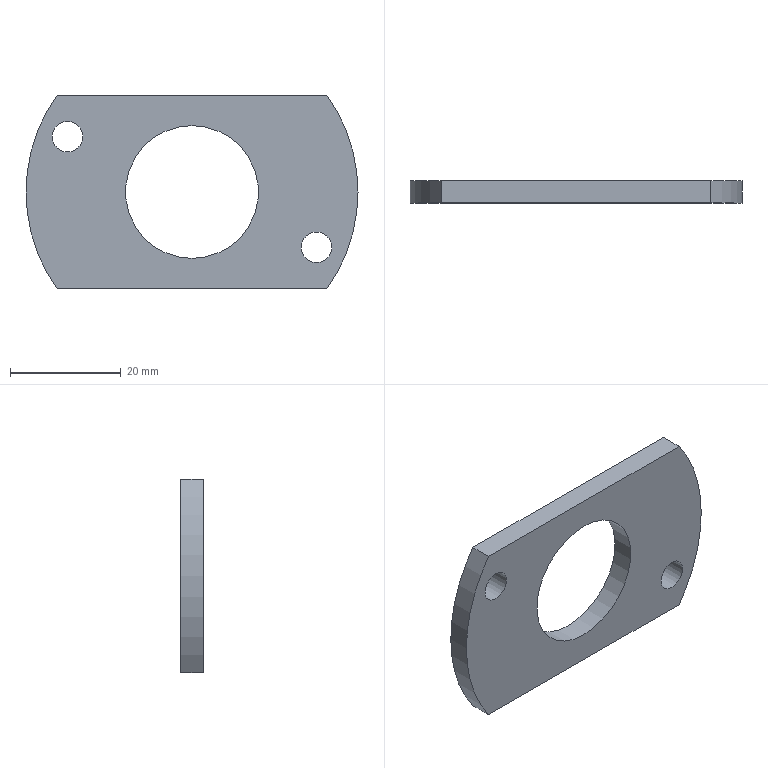Component | NX | BEARING_END_CAP_2 | 1 solid | 9 faces | box 60 x 4 x 35 mm | volume 5896 mm3 | cylinder 5 | plane 4 | commonest cylinder face diameters 60 x2 5.5 x2 24 x1
STEP:
#1=CARTESIAN_POINT('',(0.,0.,0.));
#2=DIRECTION('',(0.,0.,1.));
#3=DIRECTION('',(1.,0.,0.));
#4=AXIS2_PLACEMENT_3D('',#1,#2,#3);
#5=CARTESIAN_POINT('',(-24.367,-161.,52.5));
#6=VERTEX_POINT('',#5);
#7=CARTESIAN_POINT('',(-24.367,-161.,17.5));
#8=VERTEX_POINT('',#7);
#9=CARTESIAN_POINT('',(-0.,-161.,35.));
#10=DIRECTION('',(0.,-1.,0.));
#11=DIRECTION('',(1.,0.,0.));
#12=AXIS2_PLACEMENT_3D('',#9,#10,#11);
#13=CIRCLE('',#12,30.);
#14=CARTESIAN_POINT('',(-0.,-165.,35.));
#15=DIRECTION('',(0.,1.,0.));
#16=DIRECTION('',(0.,0.,1.));
#17=AXIS2_PLACEMENT_3D('',#14,#15,#16);
#18=CYLINDRICAL_SURFACE('',#17,30.);
#19=CARTESIAN_POINT('',(7.854,4.));
#20=DIRECTION('',(-1.,0.));
#21=VECTOR('',#20,1.);
#22=LINE('',#19,#21);
#23=(GEOMETRIC_REPRESENTATION_CONTEXT(2)PARAMETRIC_REPRESENTATION_CONTEXT()REPRESENTATION_CONTEXT('',''));
#24=DEFINITIONAL_REPRESENTATION('',(#22),#23);
#25=PCURVE('',#18,#24);
#26=CARTESIAN_POINT('',(-0.,-161.,35.));
#27=DIRECTION('',(0.,-1.,0.));
#28=DIRECTION('',(0.,0.,-1.));
#29=AXIS2_PLACEMENT_3D('',#26,#27,#28);
#30=PLANE('',#29);
#31=CARTESIAN_POINT('',(0.,0.));
#32=DIRECTION('',(0.,1.));
#33=AXIS2_PLACEMENT_2D('',#31,#32);
#34=CIRCLE('',#33,30.);
#35=(GEOMETRIC_REPRESENTATION_CONTEXT(2)PARAMETRIC_REPRESENTATION_CONTEXT()REPRESENTATION_CONTEXT('',''));
#36=DEFINITIONAL_REPRESENTATION('',(#34),#35);
#37=PCURVE('',#30,#36);
#38=SURFACE_CURVE('',#13,(#25,#37),.PCURVE_S1.);
#39=EDGE_CURVE('',#6,#8,#38,.T.);
#40=ORIENTED_EDGE('',*,*,#39,.T.);
#41=CARTESIAN_POINT('',(-24.367,-165.,17.5));
#42=VERTEX_POINT('',#41);
#43=CARTESIAN_POINT('',(-24.367,-165.,17.5));
#44=DIRECTION('',(0.,1.,0.));
#45=VECTOR('',#44,1.);
#46=LINE('',#43,#45);
#47=CARTESIAN_POINT('',(4.09,0.));
#48=DIRECTION('',(0.,1.));
#49=VECTOR('',#48,1.);
#50=LINE('',#47,#49);
#51=(GEOMETRIC_REPRESENTATION_CONTEXT(2)PARAMETRIC_REPRESENTATION_CONTEXT()REPRESENTATION_CONTEXT('',''));
#52=DEFINITIONAL_REPRESENTATION('',(#50),#51);
#53=PCURVE('',#18,#52);
#54=CARTESIAN_POINT('',(-24.367,-165.,17.5));
#55=DIRECTION('',(0.,0.,1.));
#56=DIRECTION('',(1.,0.,0.));
#57=AXIS2_PLACEMENT_3D('',#54,#55,#56);
#58=PLANE('',#57);
#59=CARTESIAN_POINT('',(0.,0.));
#60=DIRECTION('',(0.,1.));
#61=VECTOR('',#60,1.);
#62=LINE('',#59,#61);
#63=(GEOMETRIC_REPRESENTATION_CONTEXT(2)PARAMETRIC_REPRESENTATION_CONTEXT()REPRESENTATION_CONTEXT('',''));
#64=DEFINITIONAL_REPRESENTATION('',(#62),#63);
#65=PCURVE('',#58,#64);
#66=SURFACE_CURVE('',#46,(#53,#65),.PCURVE_S1.);
#67=EDGE_CURVE('',#42,#8,#66,.T.);
#68=ORIENTED_EDGE('',*,*,#67,.F.);
#69=CARTESIAN_POINT('',(-24.367,-165.,52.5));
#70=VERTEX_POINT('',#69);
#71=CARTESIAN_POINT('',(-0.,-165.,35.));
#72=DIRECTION('',(0.,-1.,0.));
#73=DIRECTION('',(1.,0.,0.));
#74=AXIS2_PLACEMENT_3D('',#71,#72,#73);
#75=CIRCLE('',#74,30.);
#76=CARTESIAN_POINT('',(7.854,0.));
#77=DIRECTION('',(-1.,0.));
#78=VECTOR('',#77,1.);
#79=LINE('',#76,#78);
#80=(GEOMETRIC_REPRESENTATION_CONTEXT(2)PARAMETRIC_REPRESENTATION_CONTEXT()REPRESENTATION_CONTEXT('',''));
#81=DEFINITIONAL_REPRESENTATION('',(#79),#80);
#82=PCURVE('',#18,#81);
#83=CARTESIAN_POINT('',(-0.,-165.,35.));
#84=DIRECTION('',(0.,-1.,0.));
#85=DIRECTION('',(0.,0.,-1.));
#86=AXIS2_PLACEMENT_3D('',#83,#84,#85);
#87=PLANE('',#86);
#88=CARTESIAN_POINT('',(0.,0.));
#89=DIRECTION('',(0.,1.));
#90=AXIS2_PLACEMENT_2D('',#88,#89);
#91=CIRCLE('',#90,30.);
#92=(GEOMETRIC_REPRESENTATION_CONTEXT(2)PARAMETRIC_REPRESENTATION_CONTEXT()REPRESENTATION_CONTEXT('',''));
#93=DEFINITIONAL_REPRESENTATION('',(#91),#92);
#94=PCURVE('',#87,#93);
#95=SURFACE_CURVE('',#75,(#82,#94),.PCURVE_S1.);
#96=EDGE_CURVE('',#70,#42,#95,.T.);
#97=ORIENTED_EDGE('',*,*,#96,.F.);
#98=CARTESIAN_POINT('',(-24.367,-165.,52.5));
#99=DIRECTION('',(0.,1.,0.));
#100=VECTOR('',#99,1.);
#101=LINE('',#98,#100);
#102=CARTESIAN_POINT('',(5.335,0.));
#103=DIRECTION('',(0.,1.));
#104=VECTOR('',#103,1.);
#105=LINE('',#102,#104);
#106=(GEOMETRIC_REPRESENTATION_CONTEXT(2)PARAMETRIC_REPRESENTATION_CONTEXT()REPRESENTATION_CONTEXT('',''));
#107=DEFINITIONAL_REPRESENTATION('',(#105),#106);
#108=PCURVE('',#18,#107);
#109=CARTESIAN_POINT('',(24.367,-165.,52.5));
#110=DIRECTION('',(0.,0.,-1.));
#111=DIRECTION('',(-1.,0.,0.));
#112=AXIS2_PLACEMENT_3D('',#109,#110,#111);
#113=PLANE('',#112);
#114=CARTESIAN_POINT('',(48.734,0.));
#115=DIRECTION('',(0.,1.));
#116=VECTOR('',#115,1.);
#117=LINE('',#114,#116);
#118=(GEOMETRIC_REPRESENTATION_CONTEXT(2)PARAMETRIC_REPRESENTATION_CONTEXT()REPRESENTATION_CONTEXT('',''));
#119=DEFINITIONAL_REPRESENTATION('',(#117),#118);
#120=PCURVE('',#113,#119);
#121=SURFACE_CURVE('',#101,(#108,#120),.PCURVE_S1.);
#122=EDGE_CURVE('',#70,#6,#121,.T.);
#123=ORIENTED_EDGE('',*,*,#122,.T.);
#124=EDGE_LOOP('',(#40,#68,#97,#123));
#125=FACE_BOUND('',#124,.T.);
#126=ADVANCED_FACE('',(#125),#18,.T.);
#127=CARTESIAN_POINT('',(24.367,-161.,17.5));
#128=VERTEX_POINT('',#127);
#129=CARTESIAN_POINT('',(-24.367,-161.,17.5));
#130=DIRECTION('',(1.,0.,0.));
#131=VECTOR('',#130,1.);
#132=LINE('',#129,#131);
#133=CARTESIAN_POINT('',(0.,4.));
#134=DIRECTION('',(1.,0.));
#135=VECTOR('',#134,1.);
#136=LINE('',#133,#135);
#137=(GEOMETRIC_REPRESENTATION_CONTEXT(2)PARAMETRIC_REPRESENTATION_CONTEXT()REPRESENTATION_CONTEXT('',''));
#138=DEFINITIONAL_REPRESENTATION('',(#136),#137);
#139=PCURVE('',#58,#138);
#140=CARTESIAN_POINT('',(17.5,-24.367));
#141=DIRECTION('',(0.,1.));
#142=VECTOR('',#141,1.);
#143=LINE('',#140,#142);
#144=(GEOMETRIC_REPRESENTATION_CONTEXT(2)PARAMETRIC_REPRESENTATION_CONTEXT()REPRESENTATION_CONTEXT('',''));
#145=DEFINITIONAL_REPRESENTATION('',(#143),#144);
#146=PCURVE('',#30,#145);
#147=SURFACE_CURVE('',#132,(#139,#146),.PCURVE_S1.);
#148=EDGE_CURVE('',#8,#128,#147,.T.);
#149=ORIENTED_EDGE('',*,*,#148,.T.);
#150=CARTESIAN_POINT('',(24.367,-165.,17.5));
#151=VERTEX_POINT('',#150);
#152=CARTESIAN_POINT('',(24.367,-165.,17.5));
#153=DIRECTION('',(0.,1.,0.));
#154=VECTOR('',#153,1.);
#155=LINE('',#152,#154);
#156=CARTESIAN_POINT('',(48.734,0.));
#157=DIRECTION('',(0.,1.));
#158=VECTOR('',#157,1.);
#159=LINE('',#156,#158);
#160=(GEOMETRIC_REPRESENTATION_CONTEXT(2)PARAMETRIC_REPRESENTATION_CONTEXT()REPRESENTATION_CONTEXT('',''));
#161=DEFINITIONAL_REPRESENTATION('',(#159),#160);
#162=PCURVE('',#58,#161);
#163=CARTESIAN_POINT('',(-0.,-165.,35.));
#164=DIRECTION('',(0.,1.,0.));
#165=DIRECTION('',(0.,0.,1.));
#166=AXIS2_PLACEMENT_3D('',#163,#164,#165);
#167=CYLINDRICAL_SURFACE('',#166,30.);
#168=CARTESIAN_POINT('',(2.194,0.));
#169=DIRECTION('',(0.,1.));
#170=VECTOR('',#169,1.);
#171=LINE('',#168,#170);
#172=(GEOMETRIC_REPRESENTATION_CONTEXT(2)PARAMETRIC_REPRESENTATION_CONTEXT()REPRESENTATION_CONTEXT('',''));
#173=DEFINITIONAL_REPRESENTATION('',(#171),#172);
#174=PCURVE('',#167,#173);
#175=SURFACE_CURVE('',#155,(#162,#174),.PCURVE_S1.);
#176=EDGE_CURVE('',#151,#128,#175,.T.);
#177=ORIENTED_EDGE('',*,*,#176,.F.);
#178=CARTESIAN_POINT('',(-24.367,-165.,17.5));
#179=DIRECTION('',(1.,0.,0.));
#180=VECTOR('',#179,1.);
#181=LINE('',#178,#180);
#182=CARTESIAN_POINT('',(0.,0.));
#183=DIRECTION('',(1.,0.));
#184=VECTOR('',#183,1.);
#185=LINE('',#182,#184);
#186=(GEOMETRIC_REPRESENTATION_CONTEXT(2)PARAMETRIC_REPRESENTATION_CONTEXT()REPRESENTATION_CONTEXT('',''));
#187=DEFINITIONAL_REPRESENTATION('',(#185),#186);
#188=PCURVE('',#58,#187);
#189=CARTESIAN_POINT('',(17.5,-24.367));
#190=DIRECTION('',(0.,1.));
#191=VECTOR('',#190,1.);
#192=LINE('',#189,#191);
#193=(GEOMETRIC_REPRESENTATION_CONTEXT(2)PARAMETRIC_REPRESENTATION_CONTEXT()REPRESENTATION_CONTEXT('',''));
#194=DEFINITIONAL_REPRESENTATION('',(#192),#193);
#195=PCURVE('',#87,#194);
#196=SURFACE_CURVE('',#181,(#188,#195),.PCURVE_S1.);
#197=EDGE_CURVE('',#42,#151,#196,.T.);
#198=ORIENTED_EDGE('',*,*,#197,.F.);
#199=ORIENTED_EDGE('',*,*,#67,.T.);
#200=EDGE_LOOP('',(#149,#177,#198,#199));
#201=FACE_BOUND('',#200,.T.);
#202=ADVANCED_FACE('',(#201),#58,.F.);
#203=CARTESIAN_POINT('',(24.367,-161.,52.5));
#204=VERTEX_POINT('',#203);
#205=CARTESIAN_POINT('',(-0.,-161.,35.));
#206=DIRECTION('',(0.,-1.,0.));
#207=DIRECTION('',(1.,0.,0.));
#208=AXIS2_PLACEMENT_3D('',#205,#206,#207);
#209=CIRCLE('',#208,30.);
#210=CARTESIAN_POINT('',(7.854,4.));
#211=DIRECTION('',(-1.,0.));
#212=VECTOR('',#211,1.);
#213=LINE('',#210,#212);
#214=(GEOMETRIC_REPRESENTATION_CONTEXT(2)PARAMETRIC_REPRESENTATION_CONTEXT()REPRESENTATION_CONTEXT('',''));
#215=DEFINITIONAL_REPRESENTATION('',(#213),#214);
#216=PCURVE('',#167,#215);
#217=CARTESIAN_POINT('',(0.,0.));
#218=DIRECTION('',(0.,1.));
#219=AXIS2_PLACEMENT_2D('',#217,#218);
#220=CIRCLE('',#219,30.);
#221=(GEOMETRIC_REPRESENTATION_CONTEXT(2)PARAMETRIC_REPRESENTATION_CONTEXT()REPRESENTATION_CONTEXT('',''));
#222=DEFINITIONAL_REPRESENTATION('',(#220),#221);
#223=PCURVE('',#30,#222);
#224=SURFACE_CURVE('',#209,(#216,#223),.PCURVE_S1.);
#225=EDGE_CURVE('',#128,#204,#224,.T.);
#226=ORIENTED_EDGE('',*,*,#225,.T.);
#227=CARTESIAN_POINT('',(24.367,-165.,52.5));
#228=VERTEX_POINT('',#227);
#229=CARTESIAN_POINT('',(24.367,-165.,52.5));
#230=DIRECTION('',(0.,1.,0.));
#231=VECTOR('',#230,1.);
#232=LINE('',#229,#231);
#233=CARTESIAN_POINT('',(0.948,0.));
#234=DIRECTION('',(0.,1.));
#235=VECTOR('',#234,1.);
#236=LINE('',#233,#235);
#237=(GEOMETRIC_REPRESENTATION_CONTEXT(2)PARAMETRIC_REPRESENTATION_CONTEXT()REPRESENTATION_CONTEXT('',''));
#238=DEFINITIONAL_REPRESENTATION('',(#236),#237);
#239=PCURVE('',#167,#238);
#240=CARTESIAN_POINT('',(-0.,0.));
#241=DIRECTION('',(0.,1.));
#242=VECTOR('',#241,1.);
#243=LINE('',#240,#242);
#244=(GEOMETRIC_REPRESENTATION_CONTEXT(2)PARAMETRIC_REPRESENTATION_CONTEXT()REPRESENTATION_CONTEXT('',''));
#245=DEFINITIONAL_REPRESENTATION('',(#243),#244);
#246=PCURVE('',#113,#245);
#247=SURFACE_CURVE('',#232,(#239,#246),.PCURVE_S1.);
#248=EDGE_CURVE('',#228,#204,#247,.T.);
#249=ORIENTED_EDGE('',*,*,#248,.F.);
#250=CARTESIAN_POINT('',(-0.,-165.,35.));
#251=DIRECTION('',(0.,-1.,0.));
#252=DIRECTION('',(1.,0.,0.));
#253=AXIS2_PLACEMENT_3D('',#250,#251,#252);
#254=CIRCLE('',#253,30.);
#255=CARTESIAN_POINT('',(7.854,0.));
#256=DIRECTION('',(-1.,0.));
#257=VECTOR('',#256,1.);
#258=LINE('',#255,#257);
#259=(GEOMETRIC_REPRESENTATION_CONTEXT(2)PARAMETRIC_REPRESENTATION_CONTEXT()REPRESENTATION_CONTEXT('',''));
#260=DEFINITIONAL_REPRESENTATION('',(#258),#259);
#261=PCURVE('',#167,#260);
#262=CARTESIAN_POINT('',(0.,0.));
#263=DIRECTION('',(0.,1.));
#264=AXIS2_PLACEMENT_2D('',#262,#263);
#265=CIRCLE('',#264,30.);
#266=(GEOMETRIC_REPRESENTATION_CONTEXT(2)PARAMETRIC_REPRESENTATION_CONTEXT()REPRESENTATION_CONTEXT('',''));
#267=DEFINITIONAL_REPRESENTATION('',(#265),#266);
#268=PCURVE('',#87,#267);
#269=SURFACE_CURVE('',#254,(#261,#268),.PCURVE_S1.);
#270=EDGE_CURVE('',#151,#228,#269,.T.);
#271=ORIENTED_EDGE('',*,*,#270,.F.);
#272=ORIENTED_EDGE('',*,*,#176,.T.);
#273=EDGE_LOOP('',(#226,#249,#271,#272));
#274=FACE_BOUND('',#273,.T.);
#275=ADVANCED_FACE('',(#274),#167,.T.);
#276=CARTESIAN_POINT('',(24.367,-161.,52.5));
#277=DIRECTION('',(-1.,0.,0.));
#278=VECTOR('',#277,1.);
#279=LINE('',#276,#278);
#280=CARTESIAN_POINT('',(0.,4.));
#281=DIRECTION('',(1.,0.));
#282=VECTOR('',#281,1.);
#283=LINE('',#280,#282);
#284=(GEOMETRIC_REPRESENTATION_CONTEXT(2)PARAMETRIC_REPRESENTATION_CONTEXT()REPRESENTATION_CONTEXT('',''));
#285=DEFINITIONAL_REPRESENTATION('',(#283),#284);
#286=PCURVE('',#113,#285);
#287=CARTESIAN_POINT('',(-17.5,24.367));
#288=DIRECTION('',(0.,-1.));
#289=VECTOR('',#288,1.);
#290=LINE('',#287,#289);
#291=(GEOMETRIC_REPRESENTATION_CONTEXT(2)PARAMETRIC_REPRESENTATION_CONTEXT()REPRESENTATION_CONTEXT('',''));
#292=DEFINITIONAL_REPRESENTATION('',(#290),#291);
#293=PCURVE('',#30,#292);
#294=SURFACE_CURVE('',#279,(#286,#293),.PCURVE_S1.);
#295=EDGE_CURVE('',#204,#6,#294,.T.);
#296=ORIENTED_EDGE('',*,*,#295,.T.);
#297=ORIENTED_EDGE('',*,*,#122,.F.);
#298=CARTESIAN_POINT('',(24.367,-165.,52.5));
#299=DIRECTION('',(-1.,0.,0.));
#300=VECTOR('',#299,1.);
#301=LINE('',#298,#300);
#302=CARTESIAN_POINT('',(0.,0.));
#303=DIRECTION('',(1.,0.));
#304=VECTOR('',#303,1.);
#305=LINE('',#302,#304);
#306=(GEOMETRIC_REPRESENTATION_CONTEXT(2)PARAMETRIC_REPRESENTATION_CONTEXT()REPRESENTATION_CONTEXT('',''));
#307=DEFINITIONAL_REPRESENTATION('',(#305),#306);
#308=PCURVE('',#113,#307);
#309=CARTESIAN_POINT('',(-17.5,24.367));
#310=DIRECTION('',(0.,-1.));
#311=VECTOR('',#310,1.);
#312=LINE('',#309,#311);
#313=(GEOMETRIC_REPRESENTATION_CONTEXT(2)PARAMETRIC_REPRESENTATION_CONTEXT()REPRESENTATION_CONTEXT('',''));
#314=DEFINITIONAL_REPRESENTATION('',(#312),#313);
#315=PCURVE('',#87,#314);
#316=SURFACE_CURVE('',#301,(#308,#315),.PCURVE_S1.);
#317=EDGE_CURVE('',#228,#70,#316,.T.);
#318=ORIENTED_EDGE('',*,*,#317,.F.);
#319=ORIENTED_EDGE('',*,*,#248,.T.);
#320=EDGE_LOOP('',(#296,#297,#318,#319));
#321=FACE_BOUND('',#320,.T.);
#322=ADVANCED_FACE('',(#321),#113,.F.);
#323=CARTESIAN_POINT('',(22.5,-165.,27.75));
#324=VERTEX_POINT('',#323);
#325=CARTESIAN_POINT('',(22.5,-165.,25.));
#326=DIRECTION('',(0.,1.,0.));
#327=DIRECTION('',(0.,0.,1.));
#328=AXIS2_PLACEMENT_3D('',#325,#326,#327);
#329=CIRCLE('',#328,2.75);
#330=CARTESIAN_POINT('',(7.25,22.5));
#331=CARTESIAN_POINT('',(7.25,27.263));
#332=CARTESIAN_POINT('',(11.375,24.882));
#333=CARTESIAN_POINT('',(15.5,22.5));
#334=CARTESIAN_POINT('',(11.375,20.118));
#335=CARTESIAN_POINT('',(7.25,17.737));
#336=CARTESIAN_POINT('',(7.25,22.5));
#337=(BOUNDED_CURVE()B_SPLINE_CURVE(2,(#330,#331,#332,#333,#334,#335,#336),.UNSPECIFIED.,.T.,.F.)B_SPLINE_CURVE_WITH_KNOTS((1,2,2,2,2,1),(-2.094,0.,2.094,4.189,6.283,8.378),.UNSPECIFIED.)CURVE()GEOMETRIC_REPRESENTATION_ITEM()RATIONAL_B_SPLINE_CURVE((1.,0.5,1.,0.5,1.,0.5,1.))REPRESENTATION_ITEM(''));
#338=(GEOMETRIC_REPRESENTATION_CONTEXT(2)PARAMETRIC_REPRESENTATION_CONTEXT()REPRESENTATION_CONTEXT('',''));
#339=DEFINITIONAL_REPRESENTATION('',(#337),#338);
#340=PCURVE('',#87,#339);
#341=CARTESIAN_POINT('',(22.5,-165.,25.));
#342=DIRECTION('',(0.,1.,0.));
#343=DIRECTION('',(0.,0.,1.));
#344=AXIS2_PLACEMENT_3D('',#341,#342,#343);
#345=CYLINDRICAL_SURFACE('',#344,2.75);
#346=CARTESIAN_POINT('',(0.,0.));
#347=DIRECTION('',(1.,0.));
#348=VECTOR('',#347,1.);
#349=LINE('',#346,#348);
#350=(GEOMETRIC_REPRESENTATION_CONTEXT(2)PARAMETRIC_REPRESENTATION_CONTEXT()REPRESENTATION_CONTEXT('',''));
#351=DEFINITIONAL_REPRESENTATION('',(#349),#350);
#352=PCURVE('',#345,#351);
#353=SURFACE_CURVE('',#329,(#340,#352),.PCURVE_S1.);
#354=EDGE_CURVE('',#324,#324,#353,.T.);
#355=ORIENTED_EDGE('',*,*,#354,.T.);
#356=EDGE_LOOP('',(#355));
#357=FACE_BOUND('',#356,.T.);
#358=CARTESIAN_POINT('',(-22.5,-165.,47.75));
#359=VERTEX_POINT('',#358);
#360=CARTESIAN_POINT('',(-22.5,-165.,45.));
#361=DIRECTION('',(0.,1.,0.));
#362=DIRECTION('',(0.,0.,1.));
#363=AXIS2_PLACEMENT_3D('',#360,#361,#362);
#364=CIRCLE('',#363,2.75);
#365=CARTESIAN_POINT('',(-12.75,-22.5));
#366=CARTESIAN_POINT('',(-12.75,-17.737));
#367=CARTESIAN_POINT('',(-8.625,-20.118));
#368=CARTESIAN_POINT('',(-4.5,-22.5));
#369=CARTESIAN_POINT('',(-8.625,-24.882));
#370=CARTESIAN_POINT('',(-12.75,-27.263));
#371=CARTESIAN_POINT('',(-12.75,-22.5));
#372=(BOUNDED_CURVE()B_SPLINE_CURVE(2,(#365,#366,#367,#368,#369,#370,#371),.UNSPECIFIED.,.T.,.F.)B_SPLINE_CURVE_WITH_KNOTS((1,2,2,2,2,1),(-2.094,0.,2.094,4.189,6.283,8.378),.UNSPECIFIED.)CURVE()GEOMETRIC_REPRESENTATION_ITEM()RATIONAL_B_SPLINE_CURVE((1.,0.5,1.,0.5,1.,0.5,1.))REPRESENTATION_ITEM(''));
#373=(GEOMETRIC_REPRESENTATION_CONTEXT(2)PARAMETRIC_REPRESENTATION_CONTEXT()REPRESENTATION_CONTEXT('',''));
#374=DEFINITIONAL_REPRESENTATION('',(#372),#373);
#375=PCURVE('',#87,#374);
#376=CARTESIAN_POINT('',(-22.5,-165.,45.));
#377=DIRECTION('',(0.,1.,0.));
#378=DIRECTION('',(0.,0.,1.));
#379=AXIS2_PLACEMENT_3D('',#376,#377,#378);
#380=CYLINDRICAL_SURFACE('',#379,2.75);
#381=CARTESIAN_POINT('',(0.,0.));
#382=DIRECTION('',(1.,0.));
#383=VECTOR('',#382,1.);
#384=LINE('',#381,#383);
#385=(GEOMETRIC_REPRESENTATION_CONTEXT(2)PARAMETRIC_REPRESENTATION_CONTEXT()REPRESENTATION_CONTEXT('',''));
#386=DEFINITIONAL_REPRESENTATION('',(#384),#385);
#387=PCURVE('',#380,#386);
#388=SURFACE_CURVE('',#364,(#375,#387),.PCURVE_S1.);
#389=EDGE_CURVE('',#359,#359,#388,.T.);
#390=ORIENTED_EDGE('',*,*,#389,.T.);
#391=EDGE_LOOP('',(#390));
#392=FACE_BOUND('',#391,.T.);
#393=CARTESIAN_POINT('',(-0.,-165.,47.));
#394=VERTEX_POINT('',#393);
#395=CARTESIAN_POINT('',(-0.,-165.,35.));
#396=DIRECTION('',(0.,1.,0.));
#397=DIRECTION('',(0.,0.,1.));
#398=AXIS2_PLACEMENT_3D('',#395,#396,#397);
#399=CIRCLE('',#398,12.);
#400=CARTESIAN_POINT('',(-12.,0.));
#401=CARTESIAN_POINT('',(-12.,20.785));
#402=CARTESIAN_POINT('',(6.,10.392));
#403=CARTESIAN_POINT('',(24.,0.));
#404=CARTESIAN_POINT('',(6.,-10.392));
#405=CARTESIAN_POINT('',(-12.,-20.785));
#406=CARTESIAN_POINT('',(-12.,0.));
#407=(BOUNDED_CURVE()B_SPLINE_CURVE(2,(#400,#401,#402,#403,#404,#405,#406),.UNSPECIFIED.,.T.,.F.)B_SPLINE_CURVE_WITH_KNOTS((1,2,2,2,2,1),(-2.094,0.,2.094,4.189,6.283,8.378),.UNSPECIFIED.)CURVE()GEOMETRIC_REPRESENTATION_ITEM()RATIONAL_B_SPLINE_CURVE((1.,0.5,1.,0.5,1.,0.5,1.))REPRESENTATION_ITEM(''));
#408=(GEOMETRIC_REPRESENTATION_CONTEXT(2)PARAMETRIC_REPRESENTATION_CONTEXT()REPRESENTATION_CONTEXT('',''));
#409=DEFINITIONAL_REPRESENTATION('',(#407),#408);
#410=PCURVE('',#87,#409);
#411=CARTESIAN_POINT('',(-0.,-165.,35.));
#412=DIRECTION('',(0.,1.,0.));
#413=DIRECTION('',(0.,0.,1.));
#414=AXIS2_PLACEMENT_3D('',#411,#412,#413);
#415=CYLINDRICAL_SURFACE('',#414,12.);
#416=CARTESIAN_POINT('',(0.,0.));
#417=DIRECTION('',(1.,0.));
#418=VECTOR('',#417,1.);
#419=LINE('',#416,#418);
#420=(GEOMETRIC_REPRESENTATION_CONTEXT(2)PARAMETRIC_REPRESENTATION_CONTEXT()REPRESENTATION_CONTEXT('',''));
#421=DEFINITIONAL_REPRESENTATION('',(#419),#420);
#422=PCURVE('',#415,#421);
#423=SURFACE_CURVE('',#399,(#410,#422),.PCURVE_S1.);
#424=EDGE_CURVE('',#394,#394,#423,.T.);
#425=ORIENTED_EDGE('',*,*,#424,.T.);
#426=EDGE_LOOP('',(#425));
#427=FACE_BOUND('',#426,.T.);
#428=ORIENTED_EDGE('',*,*,#96,.T.);
#429=ORIENTED_EDGE('',*,*,#197,.T.);
#430=ORIENTED_EDGE('',*,*,#270,.T.);
#431=ORIENTED_EDGE('',*,*,#317,.T.);
#432=EDGE_LOOP('',(#428,#429,#430,#431));
#433=FACE_BOUND('',#432,.T.);
#434=ADVANCED_FACE('',(#357,#392,#427,#433),#87,.T.);
#435=CARTESIAN_POINT('',(22.5,-161.,22.25));
#436=VERTEX_POINT('',#435);
#437=CARTESIAN_POINT('',(22.5,-161.,27.75));
#438=VERTEX_POINT('',#437);
#439=CARTESIAN_POINT('',(22.5,-161.,25.));
#440=DIRECTION('',(0.,-1.,0.));
#441=DIRECTION('',(0.,0.,-1.));
#442=AXIS2_PLACEMENT_3D('',#439,#440,#441);
#443=CIRCLE('',#442,2.75);
#444=CARTESIAN_POINT('',(10.,22.5));
#445=DIRECTION('',(1.,0.));
#446=AXIS2_PLACEMENT_2D('',#444,#445);
#447=CIRCLE('',#446,2.75);
#448=(GEOMETRIC_REPRESENTATION_CONTEXT(2)PARAMETRIC_REPRESENTATION_CONTEXT()REPRESENTATION_CONTEXT('',''));
#449=DEFINITIONAL_REPRESENTATION('',(#447),#448);
#450=PCURVE('',#30,#449);
#451=CARTESIAN_POINT('',(3.142,4.));
#452=DIRECTION('',(-1.,0.));
#453=VECTOR('',#452,1.);
#454=LINE('',#451,#453);
#455=(GEOMETRIC_REPRESENTATION_CONTEXT(2)PARAMETRIC_REPRESENTATION_CONTEXT()REPRESENTATION_CONTEXT('',''));
#456=DEFINITIONAL_REPRESENTATION('',(#454),#455);
#457=PCURVE('',#345,#456);
#458=SURFACE_CURVE('',#443,(#450,#457),.PCURVE_S1.);
#459=EDGE_CURVE('',#436,#438,#458,.T.);
#460=ORIENTED_EDGE('',*,*,#459,.T.);
#461=CARTESIAN_POINT('',(22.5,-161.,25.));
#462=DIRECTION('',(0.,-1.,0.));
#463=DIRECTION('',(0.,0.,-1.));
#464=AXIS2_PLACEMENT_3D('',#461,#462,#463);
#465=CIRCLE('',#464,2.75);
#466=CARTESIAN_POINT('',(10.,22.5));
#467=DIRECTION('',(1.,0.));
#468=AXIS2_PLACEMENT_2D('',#466,#467);
#469=CIRCLE('',#468,2.75);
#470=(GEOMETRIC_REPRESENTATION_CONTEXT(2)PARAMETRIC_REPRESENTATION_CONTEXT()REPRESENTATION_CONTEXT('',''));
#471=DEFINITIONAL_REPRESENTATION('',(#469),#470);
#472=PCURVE('',#30,#471);
#473=CARTESIAN_POINT('',(9.425,4.));
#474=DIRECTION('',(-1.,0.));
#475=VECTOR('',#474,1.);
#476=LINE('',#473,#475);
#477=(GEOMETRIC_REPRESENTATION_CONTEXT(2)PARAMETRIC_REPRESENTATION_CONTEXT()REPRESENTATION_CONTEXT('',''));
#478=DEFINITIONAL_REPRESENTATION('',(#476),#477);
#479=PCURVE('',#345,#478);
#480=SURFACE_CURVE('',#465,(#472,#479),.PCURVE_S1.);
#481=EDGE_CURVE('',#438,#436,#480,.T.);
#482=ORIENTED_EDGE('',*,*,#481,.T.);
#483=EDGE_LOOP('',(#460,#482));
#484=FACE_BOUND('',#483,.T.);
#485=CARTESIAN_POINT('',(-22.5,-161.,42.25));
#486=VERTEX_POINT('',#485);
#487=CARTESIAN_POINT('',(-22.5,-161.,47.75));
#488=VERTEX_POINT('',#487);
#489=CARTESIAN_POINT('',(-22.5,-161.,45.));
#490=DIRECTION('',(0.,-1.,0.));
#491=DIRECTION('',(0.,0.,-1.));
#492=AXIS2_PLACEMENT_3D('',#489,#490,#491);
#493=CIRCLE('',#492,2.75);
#494=CARTESIAN_POINT('',(-10.,-22.5));
#495=DIRECTION('',(1.,0.));
#496=AXIS2_PLACEMENT_2D('',#494,#495);
#497=CIRCLE('',#496,2.75);
#498=(GEOMETRIC_REPRESENTATION_CONTEXT(2)PARAMETRIC_REPRESENTATION_CONTEXT()REPRESENTATION_CONTEXT('',''));
#499=DEFINITIONAL_REPRESENTATION('',(#497),#498);
#500=PCURVE('',#30,#499);
#501=CARTESIAN_POINT('',(3.142,4.));
#502=DIRECTION('',(-1.,0.));
#503=VECTOR('',#502,1.);
#504=LINE('',#501,#503);
#505=(GEOMETRIC_REPRESENTATION_CONTEXT(2)PARAMETRIC_REPRESENTATION_CONTEXT()REPRESENTATION_CONTEXT('',''));
#506=DEFINITIONAL_REPRESENTATION('',(#504),#505);
#507=PCURVE('',#380,#506);
#508=SURFACE_CURVE('',#493,(#500,#507),.PCURVE_S1.);
#509=EDGE_CURVE('',#486,#488,#508,.T.);
#510=ORIENTED_EDGE('',*,*,#509,.T.);
#511=CARTESIAN_POINT('',(-22.5,-161.,45.));
#512=DIRECTION('',(0.,-1.,0.));
#513=DIRECTION('',(0.,0.,-1.));
#514=AXIS2_PLACEMENT_3D('',#511,#512,#513);
#515=CIRCLE('',#514,2.75);
#516=CARTESIAN_POINT('',(-10.,-22.5));
#517=DIRECTION('',(1.,0.));
#518=AXIS2_PLACEMENT_2D('',#516,#517);
#519=CIRCLE('',#518,2.75);
#520=(GEOMETRIC_REPRESENTATION_CONTEXT(2)PARAMETRIC_REPRESENTATION_CONTEXT()REPRESENTATION_CONTEXT('',''));
#521=DEFINITIONAL_REPRESENTATION('',(#519),#520);
#522=PCURVE('',#30,#521);
#523=CARTESIAN_POINT('',(9.425,4.));
#524=DIRECTION('',(-1.,0.));
#525=VECTOR('',#524,1.);
#526=LINE('',#523,#525);
#527=(GEOMETRIC_REPRESENTATION_CONTEXT(2)PARAMETRIC_REPRESENTATION_CONTEXT()REPRESENTATION_CONTEXT('',''));
#528=DEFINITIONAL_REPRESENTATION('',(#526),#527);
#529=PCURVE('',#380,#528);
#530=SURFACE_CURVE('',#515,(#522,#529),.PCURVE_S1.);
#531=EDGE_CURVE('',#488,#486,#530,.T.);
#532=ORIENTED_EDGE('',*,*,#531,.T.);
#533=EDGE_LOOP('',(#510,#532));
#534=FACE_BOUND('',#533,.T.);
#535=CARTESIAN_POINT('',(-0.,-161.,23.));
#536=VERTEX_POINT('',#535);
#537=CARTESIAN_POINT('',(-0.,-161.,47.));
#538=VERTEX_POINT('',#537);
#539=CARTESIAN_POINT('',(-0.,-161.,35.));
#540=DIRECTION('',(0.,-1.,0.));
#541=DIRECTION('',(0.,0.,-1.));
#542=AXIS2_PLACEMENT_3D('',#539,#540,#541);
#543=CIRCLE('',#542,12.);
#544=CARTESIAN_POINT('',(0.,0.));
#545=DIRECTION('',(1.,0.));
#546=AXIS2_PLACEMENT_2D('',#544,#545);
#547=CIRCLE('',#546,12.);
#548=(GEOMETRIC_REPRESENTATION_CONTEXT(2)PARAMETRIC_REPRESENTATION_CONTEXT()REPRESENTATION_CONTEXT('',''));
#549=DEFINITIONAL_REPRESENTATION('',(#547),#548);
#550=PCURVE('',#30,#549);
#551=CARTESIAN_POINT('',(3.142,4.));
#552=DIRECTION('',(-1.,0.));
#553=VECTOR('',#552,1.);
#554=LINE('',#551,#553);
#555=(GEOMETRIC_REPRESENTATION_CONTEXT(2)PARAMETRIC_REPRESENTATION_CONTEXT()REPRESENTATION_CONTEXT('',''));
#556=DEFINITIONAL_REPRESENTATION('',(#554),#555);
#557=PCURVE('',#415,#556);
#558=SURFACE_CURVE('',#543,(#550,#557),.PCURVE_S1.);
#559=EDGE_CURVE('',#536,#538,#558,.T.);
#560=ORIENTED_EDGE('',*,*,#559,.T.);
#561=CARTESIAN_POINT('',(-0.,-161.,35.));
#562=DIRECTION('',(0.,-1.,0.));
#563=DIRECTION('',(0.,0.,-1.));
#564=AXIS2_PLACEMENT_3D('',#561,#562,#563);
#565=CIRCLE('',#564,12.);
#566=CARTESIAN_POINT('',(0.,0.));
#567=DIRECTION('',(1.,0.));
#568=AXIS2_PLACEMENT_2D('',#566,#567);
#569=CIRCLE('',#568,12.);
#570=(GEOMETRIC_REPRESENTATION_CONTEXT(2)PARAMETRIC_REPRESENTATION_CONTEXT()REPRESENTATION_CONTEXT('',''));
#571=DEFINITIONAL_REPRESENTATION('',(#569),#570);
#572=PCURVE('',#30,#571);
#573=CARTESIAN_POINT('',(9.425,4.));
#574=DIRECTION('',(-1.,0.));
#575=VECTOR('',#574,1.);
#576=LINE('',#573,#575);
#577=(GEOMETRIC_REPRESENTATION_CONTEXT(2)PARAMETRIC_REPRESENTATION_CONTEXT()REPRESENTATION_CONTEXT('',''));
#578=DEFINITIONAL_REPRESENTATION('',(#576),#577);
#579=PCURVE('',#415,#578);
#580=SURFACE_CURVE('',#565,(#572,#579),.PCURVE_S1.);
#581=EDGE_CURVE('',#538,#536,#580,.T.);
#582=ORIENTED_EDGE('',*,*,#581,.T.);
#583=EDGE_LOOP('',(#560,#582));
#584=FACE_BOUND('',#583,.T.);
#585=ORIENTED_EDGE('',*,*,#39,.F.);
#586=ORIENTED_EDGE('',*,*,#295,.F.);
#587=ORIENTED_EDGE('',*,*,#225,.F.);
#588=ORIENTED_EDGE('',*,*,#148,.F.);
#589=EDGE_LOOP('',(#585,#586,#587,#588));
#590=FACE_BOUND('',#589,.T.);
#591=ADVANCED_FACE('',(#484,#534,#584,#590),#30,.F.);
#592=ORIENTED_EDGE('',*,*,#424,.T.);
#593=CARTESIAN_POINT('',(-0.,-165.,47.));
#594=CARTESIAN_POINT('',(-0.,-161.,47.));
#595=B_SPLINE_CURVE_WITH_KNOTS('',1,(#593,#594),.UNSPECIFIED.,.F.,.F.,(2,2),(0.,4.),.PIECEWISE_BEZIER_KNOTS.);
#596=CARTESIAN_POINT('',(6.283,0.));
#597=DIRECTION('',(0.,1.));
#598=VECTOR('',#597,1.);
#599=LINE('',#596,#598);
#600=(GEOMETRIC_REPRESENTATION_CONTEXT(2)PARAMETRIC_REPRESENTATION_CONTEXT()REPRESENTATION_CONTEXT('',''));
#601=DEFINITIONAL_REPRESENTATION('',(#599),#600);
#602=PCURVE('',#415,#601);
#603=CARTESIAN_POINT('',(0.,0.));
#604=DIRECTION('',(0.,1.));
#605=VECTOR('',#604,1.);
#606=LINE('',#603,#605);
#607=(GEOMETRIC_REPRESENTATION_CONTEXT(2)PARAMETRIC_REPRESENTATION_CONTEXT()REPRESENTATION_CONTEXT('',''));
#608=DEFINITIONAL_REPRESENTATION('',(#606),#607);
#609=PCURVE('',#415,#608);
#610=SEAM_CURVE('',#595,(#602,#609),.PCURVE_S1.);
#611=EDGE_CURVE('',#394,#538,#610,.T.);
#612=ORIENTED_EDGE('',*,*,#611,.T.);
#613=ORIENTED_EDGE('',*,*,#581,.T.);
#614=ORIENTED_EDGE('',*,*,#559,.T.);
#615=ORIENTED_EDGE('',*,*,#611,.F.);
#616=EDGE_LOOP('',(#592,#612,#613,#614,#615));
#617=FACE_BOUND('',#616,.F.);
#618=ADVANCED_FACE('',(#617),#415,.F.);
#619=ORIENTED_EDGE('',*,*,#389,.T.);
#620=CARTESIAN_POINT('',(-22.5,-165.,47.75));
#621=CARTESIAN_POINT('',(-22.5,-161.,47.75));
#622=B_SPLINE_CURVE_WITH_KNOTS('',1,(#620,#621),.UNSPECIFIED.,.F.,.F.,(2,2),(0.,4.),.PIECEWISE_BEZIER_KNOTS.);
#623=CARTESIAN_POINT('',(6.283,0.));
#624=DIRECTION('',(0.,1.));
#625=VECTOR('',#624,1.);
#626=LINE('',#623,#625);
#627=(GEOMETRIC_REPRESENTATION_CONTEXT(2)PARAMETRIC_REPRESENTATION_CONTEXT()REPRESENTATION_CONTEXT('',''));
#628=DEFINITIONAL_REPRESENTATION('',(#626),#627);
#629=PCURVE('',#380,#628);
#630=CARTESIAN_POINT('',(0.,0.));
#631=DIRECTION('',(0.,1.));
#632=VECTOR('',#631,1.);
#633=LINE('',#630,#632);
#634=(GEOMETRIC_REPRESENTATION_CONTEXT(2)PARAMETRIC_REPRESENTATION_CONTEXT()REPRESENTATION_CONTEXT('',''));
#635=DEFINITIONAL_REPRESENTATION('',(#633),#634);
#636=PCURVE('',#380,#635);
#637=SEAM_CURVE('',#622,(#629,#636),.PCURVE_S1.);
#638=EDGE_CURVE('',#359,#488,#637,.T.);
#639=ORIENTED_EDGE('',*,*,#638,.T.);
#640=ORIENTED_EDGE('',*,*,#531,.T.);
#641=ORIENTED_EDGE('',*,*,#509,.T.);
#642=ORIENTED_EDGE('',*,*,#638,.F.);
#643=EDGE_LOOP('',(#619,#639,#640,#641,#642));
#644=FACE_BOUND('',#643,.F.);
#645=ADVANCED_FACE('',(#644),#380,.F.);
#646=ORIENTED_EDGE('',*,*,#354,.T.);
#647=CARTESIAN_POINT('',(22.5,-165.,27.75));
#648=CARTESIAN_POINT('',(22.5,-161.,27.75));
#649=B_SPLINE_CURVE_WITH_KNOTS('',1,(#647,#648),.UNSPECIFIED.,.F.,.F.,(2,2),(0.,4.),.PIECEWISE_BEZIER_KNOTS.);
#650=CARTESIAN_POINT('',(6.283,0.));
#651=DIRECTION('',(0.,1.));
#652=VECTOR('',#651,1.);
#653=LINE('',#650,#652);
#654=(GEOMETRIC_REPRESENTATION_CONTEXT(2)PARAMETRIC_REPRESENTATION_CONTEXT()REPRESENTATION_CONTEXT('',''));
#655=DEFINITIONAL_REPRESENTATION('',(#653),#654);
#656=PCURVE('',#345,#655);
#657=CARTESIAN_POINT('',(0.,0.));
#658=DIRECTION('',(0.,1.));
#659=VECTOR('',#658,1.);
#660=LINE('',#657,#659);
#661=(GEOMETRIC_REPRESENTATION_CONTEXT(2)PARAMETRIC_REPRESENTATION_CONTEXT()REPRESENTATION_CONTEXT('',''));
#662=DEFINITIONAL_REPRESENTATION('',(#660),#661);
#663=PCURVE('',#345,#662);
#664=SEAM_CURVE('',#649,(#656,#663),.PCURVE_S1.);
#665=EDGE_CURVE('',#324,#438,#664,.T.);
#666=ORIENTED_EDGE('',*,*,#665,.T.);
#667=ORIENTED_EDGE('',*,*,#481,.T.);
#668=ORIENTED_EDGE('',*,*,#459,.T.);
#669=ORIENTED_EDGE('',*,*,#665,.F.);
#670=EDGE_LOOP('',(#646,#666,#667,#668,#669));
#671=FACE_BOUND('',#670,.F.);
#672=ADVANCED_FACE('',(#671),#345,.F.);
#673=CLOSED_SHELL('',(#126,#202,#275,#322,#434,#591,#618,#645,#672));
#674=MANIFOLD_SOLID_BREP('',#673);
#675=(LENGTH_UNIT()NAMED_UNIT(*)SI_UNIT(.MILLI.,.METRE.));
#676=UNCERTAINTY_MEASURE_WITH_UNIT(LENGTH_MEASURE(0.000002),#675,'','');
#677=(NAMED_UNIT(*)PLANE_ANGLE_UNIT()SI_UNIT($,.RADIAN.));
#678=(NAMED_UNIT(*)SI_UNIT($,.STERADIAN.)SOLID_ANGLE_UNIT());
#679=(GEOMETRIC_REPRESENTATION_CONTEXT(3)GLOBAL_UNCERTAINTY_ASSIGNED_CONTEXT((#676))GLOBAL_UNIT_ASSIGNED_CONTEXT((#675,#677,#678))REPRESENTATION_CONTEXT('',''));
#680=ADVANCED_BREP_SHAPE_REPRESENTATION('',(#4,#674),#679);